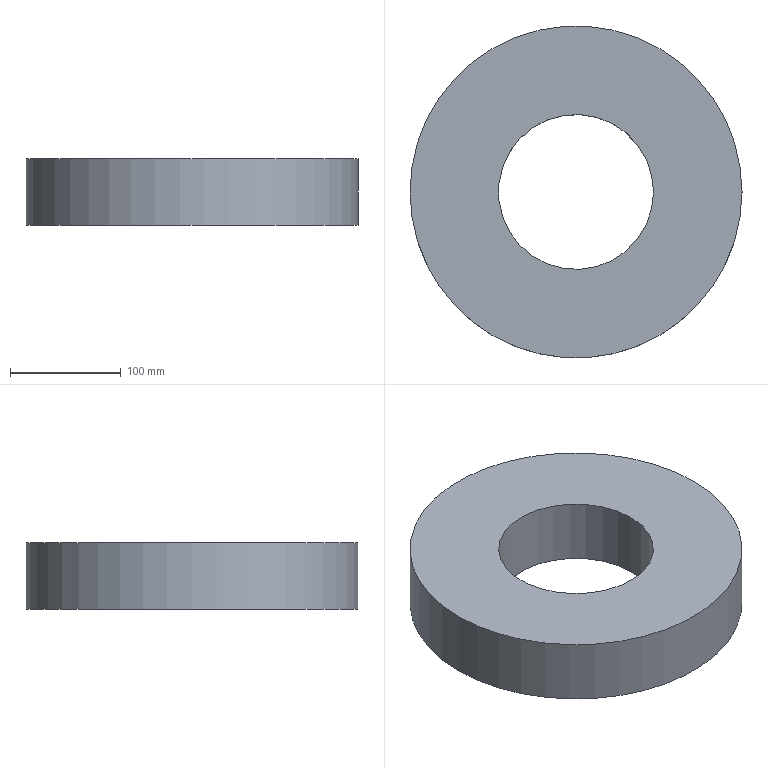Component | NX | DRAG_PLATE | 1 solid | 4 faces | box 300 x 300 x 60 mm | volume 3317522 mm3 | cylinder 2 | plane 2 | commonest cylinder face diameters 300 x1 140 x1
STEP:
#1=CARTESIAN_POINT('',(0.,0.,0.));
#2=DIRECTION('',(0.,0.,1.));
#3=DIRECTION('',(1.,0.,0.));
#4=AXIS2_PLACEMENT_3D('',#1,#2,#3);
#5=CARTESIAN_POINT('',(712.45,-0.,120.));
#6=VERTEX_POINT('',#5);
#7=CARTESIAN_POINT('',(562.45,-0.,120.));
#8=DIRECTION('',(0.,0.,-1.));
#9=DIRECTION('',(1.,0.,0.));
#10=AXIS2_PLACEMENT_3D('',#7,#8,#9);
#11=CIRCLE('',#10,150.);
#12=CARTESIAN_POINT('',(562.45,-0.,120.));
#13=DIRECTION('',(0.,0.,1.));
#14=DIRECTION('',(-1.,0.,0.));
#15=AXIS2_PLACEMENT_3D('',#12,#13,#14);
#16=CYLINDRICAL_SURFACE('',#15,150.);
#17=CARTESIAN_POINT('',(9.425,0.));
#18=DIRECTION('',(-1.,0.));
#19=VECTOR('',#18,1.);
#20=LINE('',#17,#19);
#21=(GEOMETRIC_REPRESENTATION_CONTEXT(2)PARAMETRIC_REPRESENTATION_CONTEXT()REPRESENTATION_CONTEXT('',''));
#22=DEFINITIONAL_REPRESENTATION('',(#20),#21);
#23=PCURVE('',#16,#22);
#24=CARTESIAN_POINT('',(562.45,-0.,120.));
#25=DIRECTION('',(0.,0.,-1.));
#26=DIRECTION('',(1.,0.,0.));
#27=AXIS2_PLACEMENT_3D('',#24,#25,#26);
#28=PLANE('',#27);
#29=CARTESIAN_POINT('',(0.,0.));
#30=DIRECTION('',(1.,0.));
#31=AXIS2_PLACEMENT_2D('',#29,#30);
#32=CIRCLE('',#31,150.);
#33=(GEOMETRIC_REPRESENTATION_CONTEXT(2)PARAMETRIC_REPRESENTATION_CONTEXT()REPRESENTATION_CONTEXT('',''));
#34=DEFINITIONAL_REPRESENTATION('',(#32),#33);
#35=PCURVE('',#28,#34);
#36=SURFACE_CURVE('',#11,(#23,#35),.PCURVE_S1.);
#37=EDGE_CURVE('',#6,#6,#36,.T.);
#38=ORIENTED_EDGE('',*,*,#37,.F.);
#39=CARTESIAN_POINT('',(712.45,-0.,180.));
#40=VERTEX_POINT('',#39);
#41=CARTESIAN_POINT('',(712.45,-0.,120.));
#42=CARTESIAN_POINT('',(712.45,-0.,180.));
#43=B_SPLINE_CURVE_WITH_KNOTS('',1,(#41,#42),.UNSPECIFIED.,.F.,.F.,(2,2),(0.,60.),.PIECEWISE_BEZIER_KNOTS.);
#44=CARTESIAN_POINT('',(9.425,0.));
#45=DIRECTION('',(0.,1.));
#46=VECTOR('',#45,1.);
#47=LINE('',#44,#46);
#48=(GEOMETRIC_REPRESENTATION_CONTEXT(2)PARAMETRIC_REPRESENTATION_CONTEXT()REPRESENTATION_CONTEXT('',''));
#49=DEFINITIONAL_REPRESENTATION('',(#47),#48);
#50=PCURVE('',#16,#49);
#51=CARTESIAN_POINT('',(3.142,0.));
#52=DIRECTION('',(0.,1.));
#53=VECTOR('',#52,1.);
#54=LINE('',#51,#53);
#55=(GEOMETRIC_REPRESENTATION_CONTEXT(2)PARAMETRIC_REPRESENTATION_CONTEXT()REPRESENTATION_CONTEXT('',''));
#56=DEFINITIONAL_REPRESENTATION('',(#54),#55);
#57=PCURVE('',#16,#56);
#58=SEAM_CURVE('',#43,(#50,#57),.PCURVE_S1.);
#59=EDGE_CURVE('',#6,#40,#58,.T.);
#60=ORIENTED_EDGE('',*,*,#59,.T.);
#61=CARTESIAN_POINT('',(562.45,-0.,180.));
#62=DIRECTION('',(0.,0.,-1.));
#63=DIRECTION('',(1.,0.,0.));
#64=AXIS2_PLACEMENT_3D('',#61,#62,#63);
#65=CIRCLE('',#64,150.);
#66=CARTESIAN_POINT('',(9.425,60.));
#67=DIRECTION('',(-1.,0.));
#68=VECTOR('',#67,1.);
#69=LINE('',#66,#68);
#70=(GEOMETRIC_REPRESENTATION_CONTEXT(2)PARAMETRIC_REPRESENTATION_CONTEXT()REPRESENTATION_CONTEXT('',''));
#71=DEFINITIONAL_REPRESENTATION('',(#69),#70);
#72=PCURVE('',#16,#71);
#73=CARTESIAN_POINT('',(562.45,-0.,180.));
#74=DIRECTION('',(0.,0.,-1.));
#75=DIRECTION('',(1.,0.,0.));
#76=AXIS2_PLACEMENT_3D('',#73,#74,#75);
#77=PLANE('',#76);
#78=CARTESIAN_POINT('',(0.,0.));
#79=DIRECTION('',(1.,0.));
#80=AXIS2_PLACEMENT_2D('',#78,#79);
#81=CIRCLE('',#80,150.);
#82=(GEOMETRIC_REPRESENTATION_CONTEXT(2)PARAMETRIC_REPRESENTATION_CONTEXT()REPRESENTATION_CONTEXT('',''));
#83=DEFINITIONAL_REPRESENTATION('',(#81),#82);
#84=PCURVE('',#77,#83);
#85=SURFACE_CURVE('',#65,(#72,#84),.PCURVE_S1.);
#86=EDGE_CURVE('',#40,#40,#85,.T.);
#87=ORIENTED_EDGE('',*,*,#86,.T.);
#88=ORIENTED_EDGE('',*,*,#59,.F.);
#89=EDGE_LOOP('',(#38,#60,#87,#88));
#90=FACE_BOUND('',#89,.T.);
#91=ADVANCED_FACE('',(#90),#16,.T.);
#92=CARTESIAN_POINT('',(632.45,-0.,120.));
#93=VERTEX_POINT('',#92);
#94=CARTESIAN_POINT('',(562.45,-0.,120.));
#95=DIRECTION('',(0.,0.,-1.));
#96=DIRECTION('',(1.,0.,0.));
#97=AXIS2_PLACEMENT_3D('',#94,#95,#96);
#98=CIRCLE('',#97,70.);
#99=CARTESIAN_POINT('',(562.45,-0.,120.));
#100=DIRECTION('',(0.,0.,1.));
#101=DIRECTION('',(-1.,0.,0.));
#102=AXIS2_PLACEMENT_3D('',#99,#100,#101);
#103=CYLINDRICAL_SURFACE('',#102,70.);
#104=CARTESIAN_POINT('',(9.425,0.));
#105=DIRECTION('',(-1.,0.));
#106=VECTOR('',#105,1.);
#107=LINE('',#104,#106);
#108=(GEOMETRIC_REPRESENTATION_CONTEXT(2)PARAMETRIC_REPRESENTATION_CONTEXT()REPRESENTATION_CONTEXT('',''));
#109=DEFINITIONAL_REPRESENTATION('',(#107),#108);
#110=PCURVE('',#103,#109);
#111=CARTESIAN_POINT('',(0.,0.));
#112=DIRECTION('',(1.,0.));
#113=AXIS2_PLACEMENT_2D('',#111,#112);
#114=CIRCLE('',#113,70.);
#115=(GEOMETRIC_REPRESENTATION_CONTEXT(2)PARAMETRIC_REPRESENTATION_CONTEXT()REPRESENTATION_CONTEXT('',''));
#116=DEFINITIONAL_REPRESENTATION('',(#114),#115);
#117=PCURVE('',#28,#116);
#118=SURFACE_CURVE('',#98,(#110,#117),.PCURVE_S1.);
#119=EDGE_CURVE('',#93,#93,#118,.T.);
#120=ORIENTED_EDGE('',*,*,#119,.F.);
#121=CARTESIAN_POINT('',(632.45,-0.,180.));
#122=VERTEX_POINT('',#121);
#123=CARTESIAN_POINT('',(632.45,-0.,120.));
#124=CARTESIAN_POINT('',(632.45,-0.,180.));
#125=B_SPLINE_CURVE_WITH_KNOTS('',1,(#123,#124),.UNSPECIFIED.,.F.,.F.,(2,2),(0.,60.),.PIECEWISE_BEZIER_KNOTS.);
#126=CARTESIAN_POINT('',(9.425,0.));
#127=DIRECTION('',(0.,1.));
#128=VECTOR('',#127,1.);
#129=LINE('',#126,#128);
#130=(GEOMETRIC_REPRESENTATION_CONTEXT(2)PARAMETRIC_REPRESENTATION_CONTEXT()REPRESENTATION_CONTEXT('',''));
#131=DEFINITIONAL_REPRESENTATION('',(#129),#130);
#132=PCURVE('',#103,#131);
#133=CARTESIAN_POINT('',(3.142,0.));
#134=DIRECTION('',(0.,1.));
#135=VECTOR('',#134,1.);
#136=LINE('',#133,#135);
#137=(GEOMETRIC_REPRESENTATION_CONTEXT(2)PARAMETRIC_REPRESENTATION_CONTEXT()REPRESENTATION_CONTEXT('',''));
#138=DEFINITIONAL_REPRESENTATION('',(#136),#137);
#139=PCURVE('',#103,#138);
#140=SEAM_CURVE('',#125,(#132,#139),.PCURVE_S1.);
#141=EDGE_CURVE('',#93,#122,#140,.T.);
#142=ORIENTED_EDGE('',*,*,#141,.T.);
#143=CARTESIAN_POINT('',(562.45,-0.,180.));
#144=DIRECTION('',(0.,0.,-1.));
#145=DIRECTION('',(1.,0.,0.));
#146=AXIS2_PLACEMENT_3D('',#143,#144,#145);
#147=CIRCLE('',#146,70.);
#148=CARTESIAN_POINT('',(9.425,60.));
#149=DIRECTION('',(-1.,0.));
#150=VECTOR('',#149,1.);
#151=LINE('',#148,#150);
#152=(GEOMETRIC_REPRESENTATION_CONTEXT(2)PARAMETRIC_REPRESENTATION_CONTEXT()REPRESENTATION_CONTEXT('',''));
#153=DEFINITIONAL_REPRESENTATION('',(#151),#152);
#154=PCURVE('',#103,#153);
#155=CARTESIAN_POINT('',(0.,0.));
#156=DIRECTION('',(1.,0.));
#157=AXIS2_PLACEMENT_2D('',#155,#156);
#158=CIRCLE('',#157,70.);
#159=(GEOMETRIC_REPRESENTATION_CONTEXT(2)PARAMETRIC_REPRESENTATION_CONTEXT()REPRESENTATION_CONTEXT('',''));
#160=DEFINITIONAL_REPRESENTATION('',(#158),#159);
#161=PCURVE('',#77,#160);
#162=SURFACE_CURVE('',#147,(#154,#161),.PCURVE_S1.);
#163=EDGE_CURVE('',#122,#122,#162,.T.);
#164=ORIENTED_EDGE('',*,*,#163,.T.);
#165=ORIENTED_EDGE('',*,*,#141,.F.);
#166=EDGE_LOOP('',(#120,#142,#164,#165));
#167=FACE_BOUND('',#166,.F.);
#168=ADVANCED_FACE('',(#167),#103,.F.);
#169=ORIENTED_EDGE('',*,*,#37,.T.);
#170=EDGE_LOOP('',(#169));
#171=FACE_BOUND('',#170,.T.);
#172=ORIENTED_EDGE('',*,*,#119,.F.);
#173=EDGE_LOOP('',(#172));
#174=FACE_BOUND('',#173,.T.);
#175=ADVANCED_FACE('',(#171,#174),#28,.T.);
#176=ORIENTED_EDGE('',*,*,#86,.F.);
#177=EDGE_LOOP('',(#176));
#178=FACE_BOUND('',#177,.T.);
#179=ORIENTED_EDGE('',*,*,#163,.T.);
#180=EDGE_LOOP('',(#179));
#181=FACE_BOUND('',#180,.T.);
#182=ADVANCED_FACE('',(#178,#181),#77,.F.);
#183=CLOSED_SHELL('',(#91,#168,#175,#182));
#184=MANIFOLD_SOLID_BREP('',#183);
#185=(LENGTH_UNIT()NAMED_UNIT(*)SI_UNIT(.MILLI.,.METRE.));
#186=UNCERTAINTY_MEASURE_WITH_UNIT(LENGTH_MEASURE(0.00001),#185,'','');
#187=(NAMED_UNIT(*)PLANE_ANGLE_UNIT()SI_UNIT($,.RADIAN.));
#188=(NAMED_UNIT(*)SI_UNIT($,.STERADIAN.)SOLID_ANGLE_UNIT());
#189=(GEOMETRIC_REPRESENTATION_CONTEXT(3)GLOBAL_UNCERTAINTY_ASSIGNED_CONTEXT((#186))GLOBAL_UNIT_ASSIGNED_CONTEXT((#185,#187,#188))REPRESENTATION_CONTEXT('',''));
#190=ADVANCED_BREP_SHAPE_REPRESENTATION('',(#4,#184),#189);